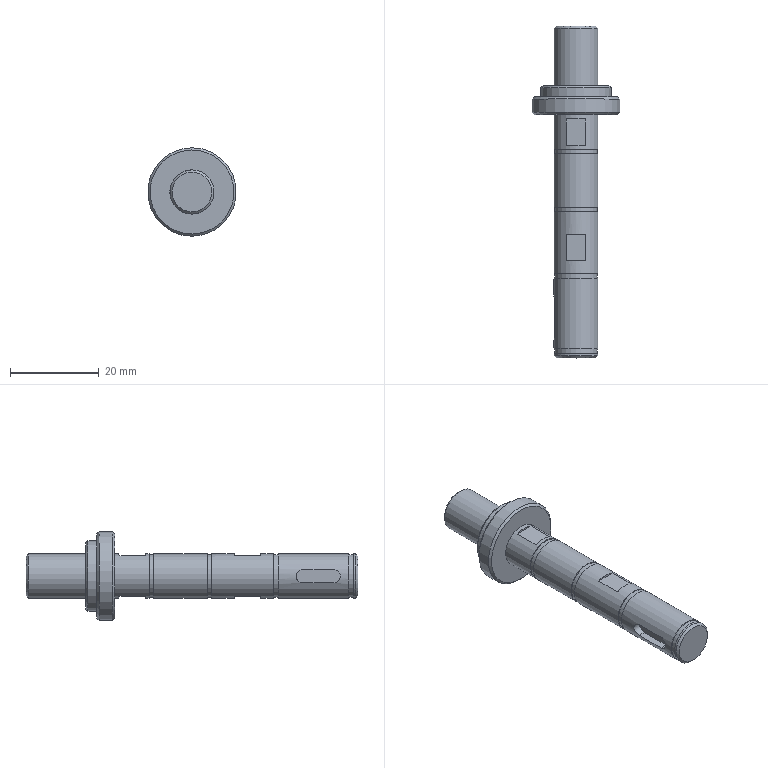Component | NX | MOUNTING_SHAFT | 1 solid | 47 faces | volume 6999 mm3 | plane 28 | cylinder 14 | cone 5 | commonest cylinder face diameters 10 x6 9.6 x4 3 x2 20 x1 16 x1